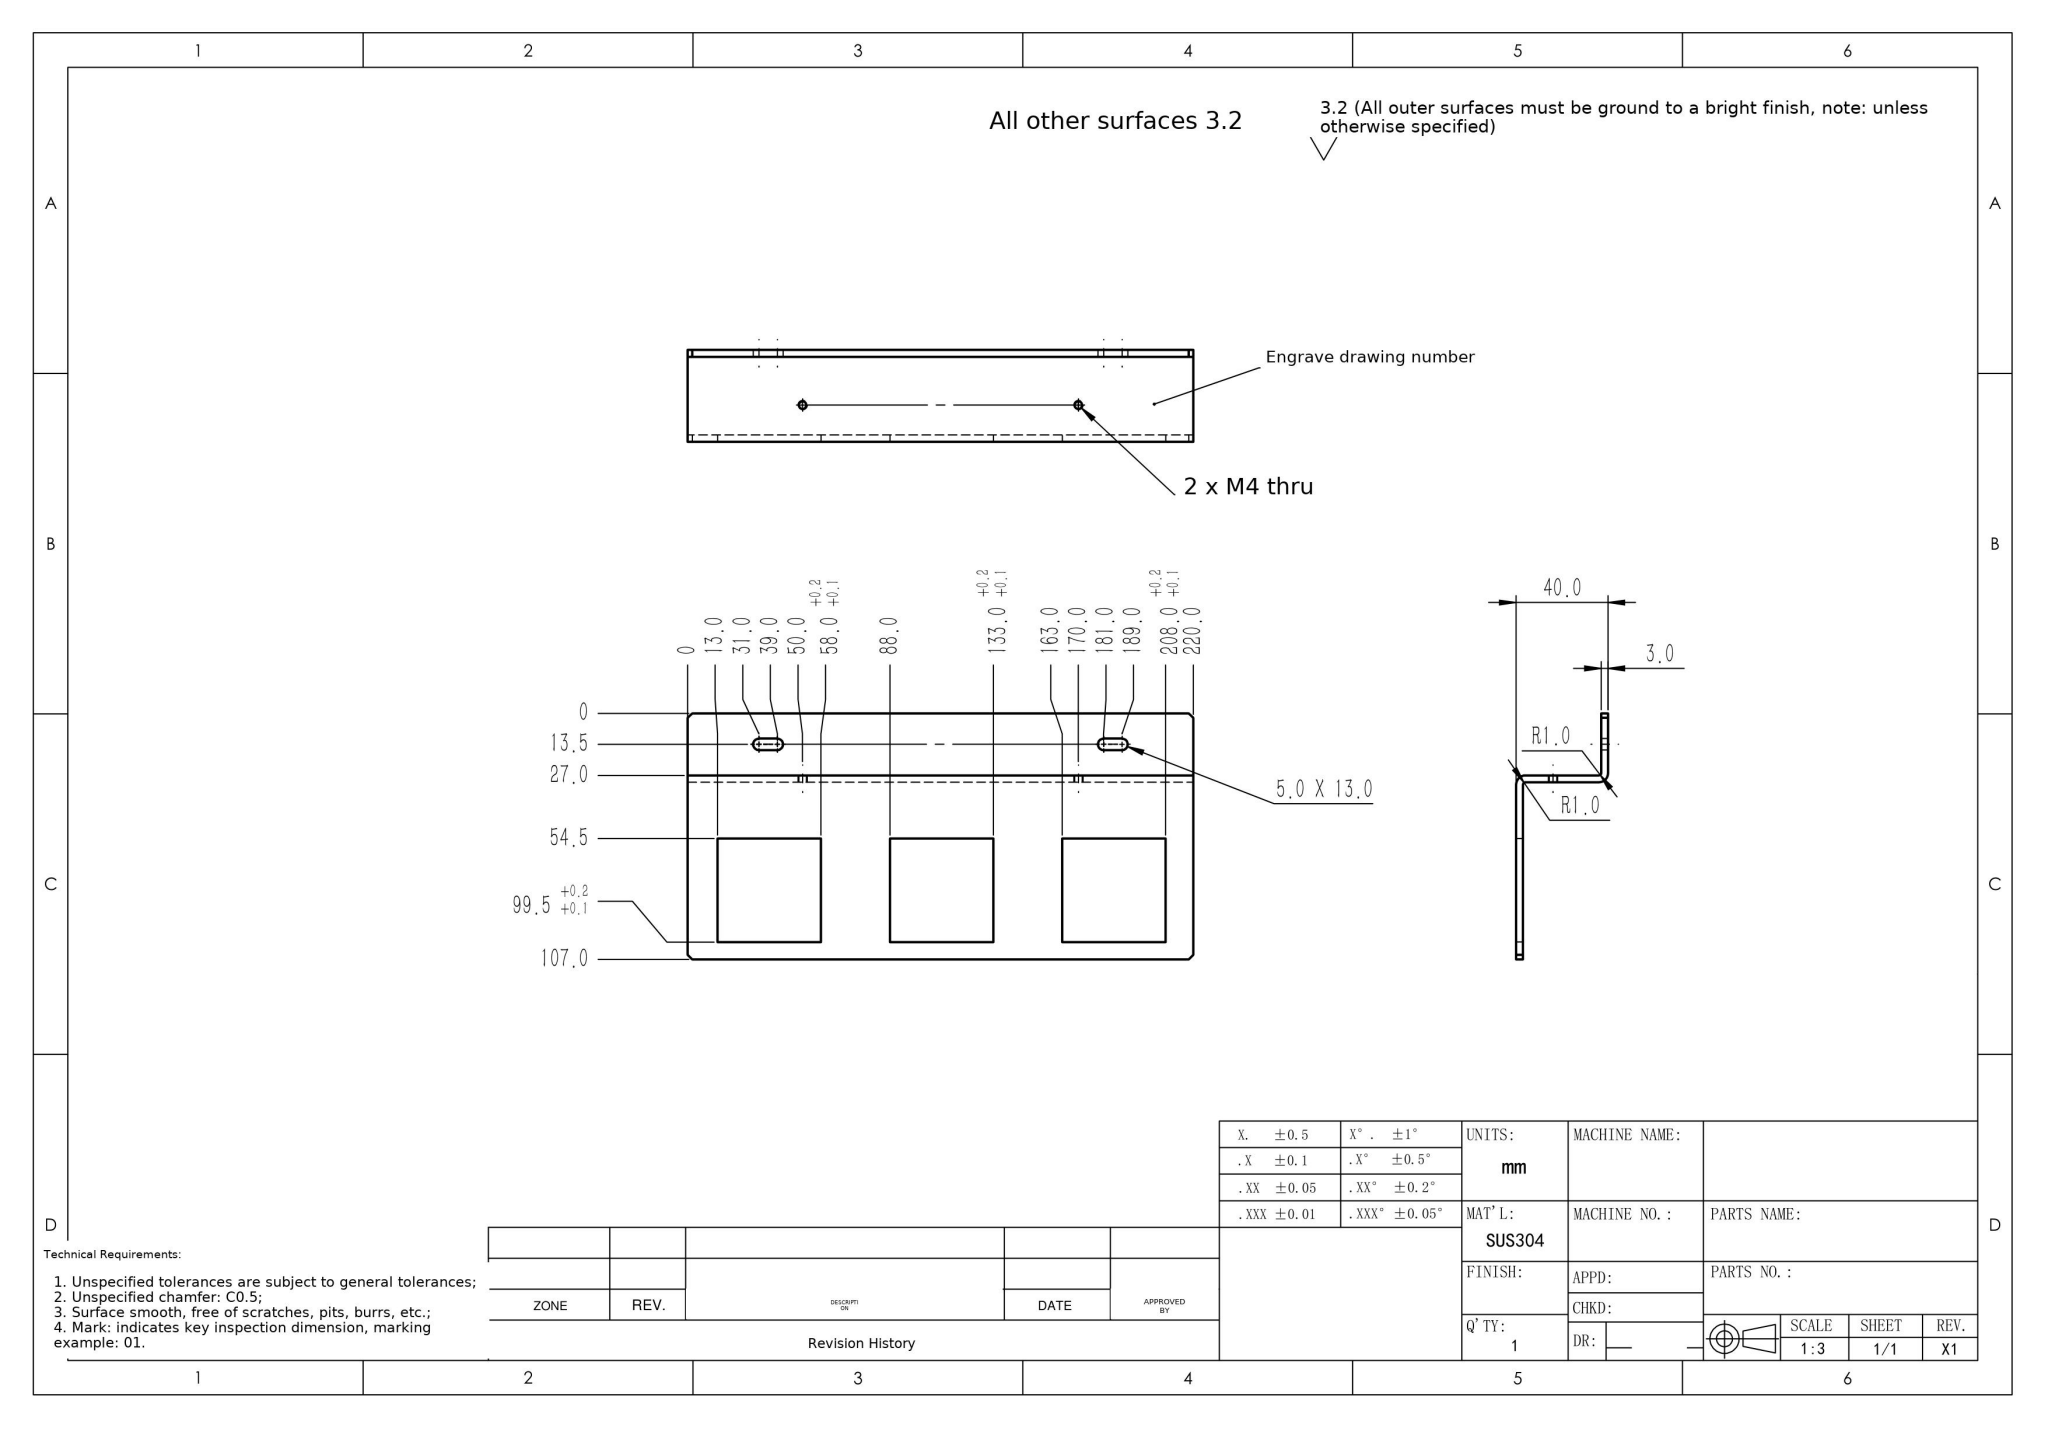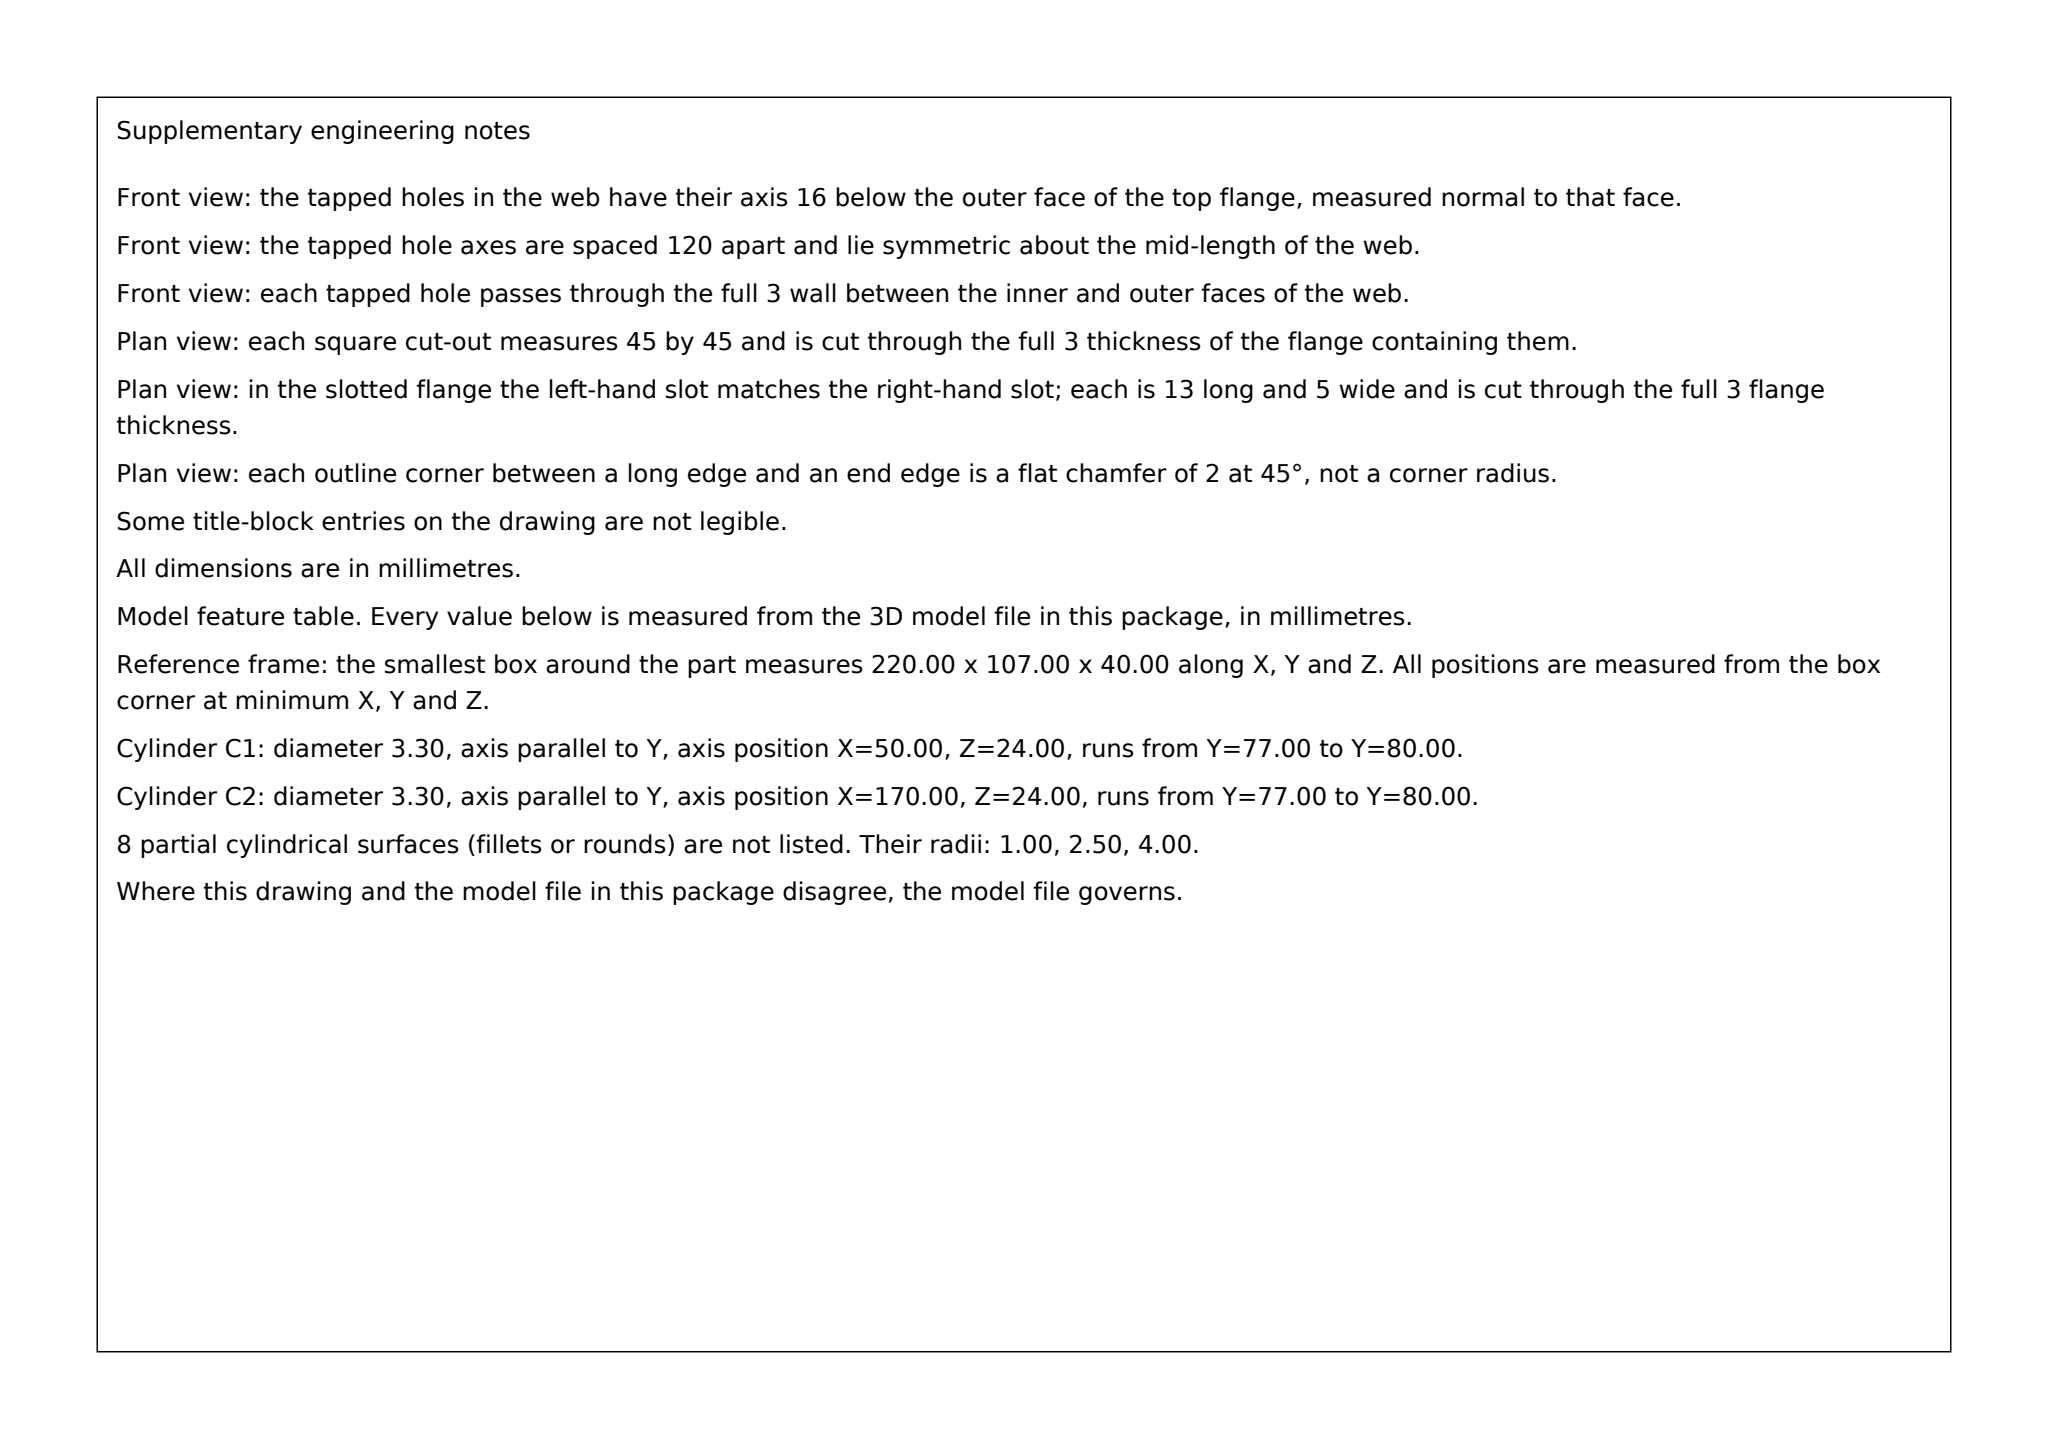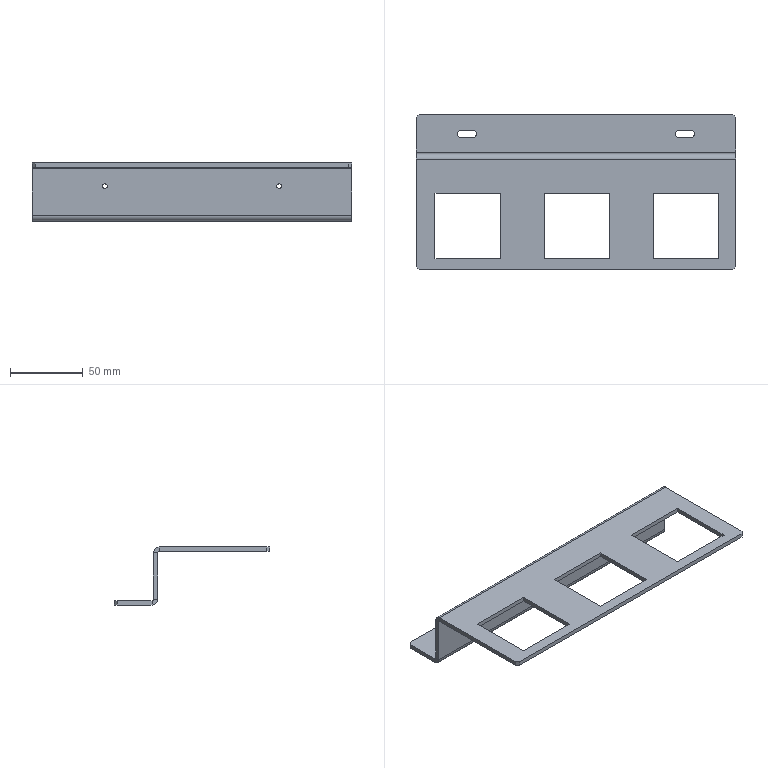Part | SolidWorks | mm | 1 solid | 52 faces | box 220 x 107 x 40 mm | volume 74966 mm3 | plane 38 | cylinder 14 | commonest cylinder face diameters 5 x6 3.3 x4 8 x2 2 x2